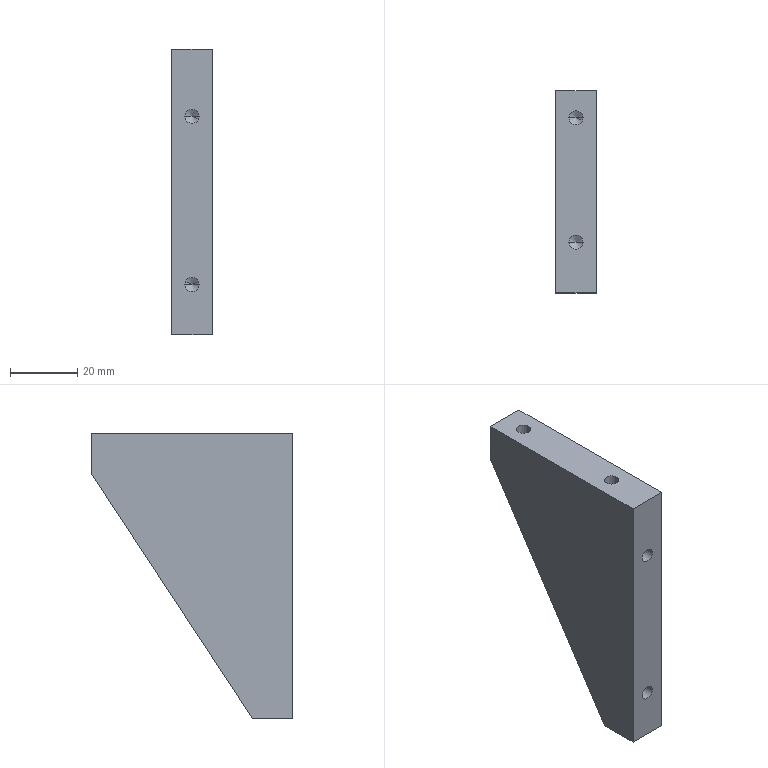Component | SolidWorks | HandlingMechanism-2_A0111-2 | 1 solid | 23 faces | box 12 x 60 x 85 mm | volume 39377 mm3 | cylinder 8 | cone 8 | plane 7 | commonest cylinder face diameters 4.2 x8
build123d program:
from build123d import *

# Parameters (mm, degrees)
SKETCH1_W             = 85
SKETCH1_H             = 60
BOSS_EXTRUDE1_DEPTH   = 6
CUT_EXTRUDE1_DEPTH    = 12
M5_TAPPED_HOLE1_D     = 4.2
M5_TAPPED_HOLE1_DEPTH = 14
M5_TAPPED_HOLE1_TIP   = 1.262
M5_TAPPED_HOLE2_D     = 4.2
M5_TAPPED_HOLE2_DEPTH = 14
M5_TAPPED_HOLE2_TIP   = 1.262


with BuildPart() as part:
    # Sketch1 → Boss-Extrude1 (new, symmetric)
    with BuildSketch(Plane.XY):
        Rectangle(SKETCH1_W, SKETCH1_H)
    extrude(amount=BOSS_EXTRUDE1_DEPTH, both=True)

    # Sketch2 → Cut-Extrude1 (cut)
    with BuildSketch(Plane.XY.offset(6)):
        Polygon((-42.5, -18), (30.5, 30), (-42.5, 30), align=None)
    extrude(amount=-CUT_EXTRUDE1_DEPTH, mode=Mode.SUBTRACT)

    # M5 Tapped Hole1
    with Locations(Plane(origin=(0, -30, 0), x_dir=(-1, 0, 0), z_dir=(0, -1, 0))):
        with Locations((27.5, 0), (-22.5, 0)):
            Hole(M5_TAPPED_HOLE1_D / 2, depth=M5_TAPPED_HOLE1_DEPTH)
            with Locations((0, 0, -(M5_TAPPED_HOLE1_DEPTH + M5_TAPPED_HOLE1_TIP / 2))):  # 118° drill point
                Cone(0, M5_TAPPED_HOLE1_D / 2, M5_TAPPED_HOLE1_TIP, mode=Mode.SUBTRACT)

    # M5 Tapped Hole2
    with Locations(Plane(origin=(42.5, 0, 0), x_dir=(0, 0, -1), z_dir=(1, 0, 0))):
        with Locations((0, 22), (0, -15)):
            Hole(M5_TAPPED_HOLE2_D / 2, depth=M5_TAPPED_HOLE2_DEPTH)
            with Locations((0, 0, -(M5_TAPPED_HOLE2_DEPTH + M5_TAPPED_HOLE2_TIP / 2))):  # 118° drill point
                Cone(0, M5_TAPPED_HOLE2_D / 2, M5_TAPPED_HOLE2_TIP, mode=Mode.SUBTRACT)


solid = part.part

# Placed as in the assembly
solid = solid.moved(Location((25.881, 81.5, 80.5), (0, -90, 0)))
STEP:
#1=COLOUR_RGB('',0.7922,0.8196,0.9333);
#2=FILL_AREA_STYLE_COLOUR('',#1);
#3=FILL_AREA_STYLE('',(#2));
#4=SURFACE_STYLE_FILL_AREA(#3);
#5=SURFACE_SIDE_STYLE('',(#4));
#6=SURFACE_STYLE_USAGE(.BOTH.,#5);
#7=PRESENTATION_STYLE_ASSIGNMENT((#6));
#8=CARTESIAN_POINT('',(0.9362,4.075,4.291));
#9=VERTEX_POINT('',#8);
#10=CARTESIAN_POINT('',(1.102,4.075,4.291));
#11=VERTEX_POINT('',#10);
#12=CARTESIAN_POINT('',(1.019,4.075,4.291));
#13=DIRECTION('',(0.,-0.,1.));
#14=DIRECTION('',(1.,0.,-0.));
#15=AXIS2_PLACEMENT_3D('',#12,#13,#14);
#16=CIRCLE('',#15,0.08268);
#17=EDGE_CURVE('',#9,#11,#16,.T.);
#18=ORIENTED_EDGE('',*,*,#17,.F.);
#19=CARTESIAN_POINT('',(0.9362,4.075,4.843));
#20=VERTEX_POINT('',#19);
#21=CARTESIAN_POINT('',(0.9362,4.075,4.843));
#22=DIRECTION('',(0.,-0.,1.));
#23=VECTOR('',#22,39.37);
#24=LINE('',#21,#23);
#25=EDGE_CURVE('',#9,#20,#24,.T.);
#26=ORIENTED_EDGE('',*,*,#25,.T.);
#27=CARTESIAN_POINT('',(1.102,4.075,4.843));
#28=VERTEX_POINT('',#27);
#29=CARTESIAN_POINT('',(1.019,4.075,4.843));
#30=DIRECTION('',(0.,-0.,1.));
#31=DIRECTION('',(1.,0.,-0.));
#32=AXIS2_PLACEMENT_3D('',#29,#30,#31);
#33=CIRCLE('',#32,0.08268);
#34=EDGE_CURVE('',#20,#28,#33,.T.);
#35=ORIENTED_EDGE('',*,*,#34,.T.);
#36=CARTESIAN_POINT('',(1.102,4.075,4.843));
#37=DIRECTION('',(0.,-0.,1.));
#38=VECTOR('',#37,39.37);
#39=LINE('',#36,#38);
#40=EDGE_CURVE('',#11,#28,#39,.T.);
#41=ORIENTED_EDGE('',*,*,#40,.F.);
#42=EDGE_LOOP('',(#18,#26,#35,#41));
#43=FACE_OUTER_BOUND('',#42,.T.);
#44=CARTESIAN_POINT('',(1.019,4.075,4.843));
#45=DIRECTION('',(0.,-0.,1.));
#46=DIRECTION('',(1.,0.,-0.));
#47=AXIS2_PLACEMENT_3D('',#44,#45,#46);
#48=CYLINDRICAL_SURFACE('',#47,0.08268);
#49=ADVANCED_FACE('',(#43),#48,.F.);
#50=CARTESIAN_POINT('',(1.019,4.075,4.242));
#51=VERTEX_POINT('',#50);
#52=CARTESIAN_POINT('',(1.102,4.075,4.291));
#53=DIRECTION('',(0.8572,0.,0.515));
#54=VECTOR('',#53,39.37);
#55=LINE('',#52,#54);
#56=EDGE_CURVE('',#51,#11,#55,.T.);
#57=ORIENTED_EDGE('',*,*,#56,.F.);
#58=CARTESIAN_POINT('',(0.9362,4.075,4.291));
#59=DIRECTION('',(-0.8572,-0.,0.515));
#60=VECTOR('',#59,39.37);
#61=LINE('',#58,#60);
#62=EDGE_CURVE('',#51,#9,#61,.T.);
#63=ORIENTED_EDGE('',*,*,#62,.T.);
#64=ORIENTED_EDGE('',*,*,#17,.T.);
#65=EDGE_LOOP('',(#57,#63,#64));
#66=FACE_OUTER_BOUND('',#65,.T.);
#67=CARTESIAN_POINT('',(1.019,4.075,4.291));
#68=DIRECTION('',(0.,-0.,1.));
#69=DIRECTION('',(1.,0.,-0.));
#70=AXIS2_PLACEMENT_3D('',#67,#68,#69);
#71=CONICAL_SURFACE('',#70,0.08268,1.03);
#72=ADVANCED_FACE('',(#66),#71,.F.);
#73=CARTESIAN_POINT('',(0.9362,2.618,4.291));
#74=VERTEX_POINT('',#73);
#75=CARTESIAN_POINT('',(1.102,2.618,4.291));
#76=VERTEX_POINT('',#75);
#77=CARTESIAN_POINT('',(1.019,2.618,4.291));
#78=DIRECTION('',(0.,-0.,1.));
#79=DIRECTION('',(1.,0.,-0.));
#80=AXIS2_PLACEMENT_3D('',#77,#78,#79);
#81=CIRCLE('',#80,0.08268);
#82=EDGE_CURVE('',#74,#76,#81,.T.);
#83=ORIENTED_EDGE('',*,*,#82,.F.);
#84=CARTESIAN_POINT('',(0.9362,2.618,4.843));
#85=VERTEX_POINT('',#84);
#86=CARTESIAN_POINT('',(0.9362,2.618,4.843));
#87=DIRECTION('',(0.,-0.,1.));
#88=VECTOR('',#87,39.37);
#89=LINE('',#86,#88);
#90=EDGE_CURVE('',#74,#85,#89,.T.);
#91=ORIENTED_EDGE('',*,*,#90,.T.);
#92=CARTESIAN_POINT('',(1.102,2.618,4.843));
#93=VERTEX_POINT('',#92);
#94=CARTESIAN_POINT('',(1.019,2.618,4.843));
#95=DIRECTION('',(0.,-0.,1.));
#96=DIRECTION('',(1.,0.,-0.));
#97=AXIS2_PLACEMENT_3D('',#94,#95,#96);
#98=CIRCLE('',#97,0.08268);
#99=EDGE_CURVE('',#85,#93,#98,.T.);
#100=ORIENTED_EDGE('',*,*,#99,.T.);
#101=CARTESIAN_POINT('',(1.102,2.618,4.843));
#102=DIRECTION('',(0.,-0.,1.));
#103=VECTOR('',#102,39.37);
#104=LINE('',#101,#103);
#105=EDGE_CURVE('',#76,#93,#104,.T.);
#106=ORIENTED_EDGE('',*,*,#105,.F.);
#107=EDGE_LOOP('',(#83,#91,#100,#106));
#108=FACE_OUTER_BOUND('',#107,.T.);
#109=CARTESIAN_POINT('',(1.019,2.618,4.843));
#110=DIRECTION('',(0.,-0.,1.));
#111=DIRECTION('',(1.,0.,-0.));
#112=AXIS2_PLACEMENT_3D('',#109,#110,#111);
#113=CYLINDRICAL_SURFACE('',#112,0.08268);
#114=ADVANCED_FACE('',(#108),#113,.F.);
#115=CARTESIAN_POINT('',(1.019,2.618,4.242));
#116=VERTEX_POINT('',#115);
#117=CARTESIAN_POINT('',(1.102,2.618,4.291));
#118=DIRECTION('',(0.8572,0.,0.515));
#119=VECTOR('',#118,39.37);
#120=LINE('',#117,#119);
#121=EDGE_CURVE('',#116,#76,#120,.T.);
#122=ORIENTED_EDGE('',*,*,#121,.F.);
#123=CARTESIAN_POINT('',(0.9362,2.618,4.291));
#124=DIRECTION('',(-0.8572,-0.,0.515));
#125=VECTOR('',#124,39.37);
#126=LINE('',#123,#125);
#127=EDGE_CURVE('',#116,#74,#126,.T.);
#128=ORIENTED_EDGE('',*,*,#127,.T.);
#129=ORIENTED_EDGE('',*,*,#82,.T.);
#130=EDGE_LOOP('',(#122,#128,#129));
#131=FACE_OUTER_BOUND('',#130,.T.);
#132=CARTESIAN_POINT('',(1.019,2.618,4.291));
#133=DIRECTION('',(0.,-0.,1.));
#134=DIRECTION('',(1.,0.,-0.));
#135=AXIS2_PLACEMENT_3D('',#132,#133,#134);
#136=CONICAL_SURFACE('',#135,0.08268,1.03);
#137=ADVANCED_FACE('',(#131),#136,.F.);
#138=CARTESIAN_POINT('',(0.9362,2.579,2.087));
#139=VERTEX_POINT('',#138);
#140=CARTESIAN_POINT('',(1.102,2.579,2.087));
#141=VERTEX_POINT('',#140);
#142=CARTESIAN_POINT('',(1.019,2.579,2.087));
#143=DIRECTION('',(0.,-1.,-0.));
#144=DIRECTION('',(1.,0.,-0.));
#145=AXIS2_PLACEMENT_3D('',#142,#143,#144);
#146=CIRCLE('',#145,0.08268);
#147=EDGE_CURVE('',#139,#141,#146,.T.);
#148=ORIENTED_EDGE('',*,*,#147,.F.);
#149=CARTESIAN_POINT('',(0.9362,2.028,2.087));
#150=VERTEX_POINT('',#149);
#151=CARTESIAN_POINT('',(0.9362,2.028,2.087));
#152=DIRECTION('',(0.,-1.,-0.));
#153=VECTOR('',#152,39.37);
#154=LINE('',#151,#153);
#155=EDGE_CURVE('',#139,#150,#154,.T.);
#156=ORIENTED_EDGE('',*,*,#155,.T.);
#157=CARTESIAN_POINT('',(1.102,2.028,2.087));
#158=VERTEX_POINT('',#157);
#159=CARTESIAN_POINT('',(1.019,2.028,2.087));
#160=DIRECTION('',(0.,-1.,-0.));
#161=DIRECTION('',(1.,0.,-0.));
#162=AXIS2_PLACEMENT_3D('',#159,#160,#161);
#163=CIRCLE('',#162,0.08268);
#164=EDGE_CURVE('',#150,#158,#163,.T.);
#165=ORIENTED_EDGE('',*,*,#164,.T.);
#166=CARTESIAN_POINT('',(1.102,2.028,2.087));
#167=DIRECTION('',(0.,-1.,-0.));
#168=VECTOR('',#167,39.37);
#169=LINE('',#166,#168);
#170=EDGE_CURVE('',#141,#158,#169,.T.);
#171=ORIENTED_EDGE('',*,*,#170,.F.);
#172=EDGE_LOOP('',(#148,#156,#165,#171));
#173=FACE_OUTER_BOUND('',#172,.T.);
#174=CARTESIAN_POINT('',(1.019,2.028,2.087));
#175=DIRECTION('',(0.,-1.,-0.));
#176=DIRECTION('',(1.,0.,-0.));
#177=AXIS2_PLACEMENT_3D('',#174,#175,#176);
#178=CYLINDRICAL_SURFACE('',#177,0.08268);
#179=ADVANCED_FACE('',(#173),#178,.F.);
#180=CARTESIAN_POINT('',(1.019,2.628,2.087));
#181=VERTEX_POINT('',#180);
#182=CARTESIAN_POINT('',(1.102,2.579,2.087));
#183=DIRECTION('',(0.8572,-0.515,-0.));
#184=VECTOR('',#183,39.37);
#185=LINE('',#182,#184);
#186=EDGE_CURVE('',#181,#141,#185,.T.);
#187=ORIENTED_EDGE('',*,*,#186,.F.);
#188=CARTESIAN_POINT('',(0.9362,2.579,2.087));
#189=DIRECTION('',(-0.8572,-0.515,0.));
#190=VECTOR('',#189,39.37);
#191=LINE('',#188,#190);
#192=EDGE_CURVE('',#181,#139,#191,.T.);
#193=ORIENTED_EDGE('',*,*,#192,.T.);
#194=ORIENTED_EDGE('',*,*,#147,.T.);
#195=EDGE_LOOP('',(#187,#193,#194));
#196=FACE_OUTER_BOUND('',#195,.T.);
#197=CARTESIAN_POINT('',(1.019,2.579,2.087));
#198=DIRECTION('',(0.,-1.,-0.));
#199=DIRECTION('',(1.,0.,-0.));
#200=AXIS2_PLACEMENT_3D('',#197,#198,#199);
#201=CONICAL_SURFACE('',#200,0.08268,1.03);
#202=ADVANCED_FACE('',(#196),#201,.F.);
#203=CARTESIAN_POINT('',(0.9362,2.579,4.055));
#204=VERTEX_POINT('',#203);
#205=CARTESIAN_POINT('',(1.102,2.579,4.055));
#206=VERTEX_POINT('',#205);
#207=CARTESIAN_POINT('',(1.019,2.579,4.055));
#208=DIRECTION('',(0.,-1.,-0.));
#209=DIRECTION('',(1.,0.,-0.));
#210=AXIS2_PLACEMENT_3D('',#207,#208,#209);
#211=CIRCLE('',#210,0.08268);
#212=EDGE_CURVE('',#204,#206,#211,.T.);
#213=ORIENTED_EDGE('',*,*,#212,.F.);
#214=CARTESIAN_POINT('',(0.9362,2.028,4.055));
#215=VERTEX_POINT('',#214);
#216=CARTESIAN_POINT('',(0.9362,2.028,4.055));
#217=DIRECTION('',(0.,-1.,-0.));
#218=VECTOR('',#217,39.37);
#219=LINE('',#216,#218);
#220=EDGE_CURVE('',#204,#215,#219,.T.);
#221=ORIENTED_EDGE('',*,*,#220,.T.);
#222=CARTESIAN_POINT('',(1.102,2.028,4.055));
#223=VERTEX_POINT('',#222);
#224=CARTESIAN_POINT('',(1.019,2.028,4.055));
#225=DIRECTION('',(0.,-1.,-0.));
#226=DIRECTION('',(1.,0.,-0.));
#227=AXIS2_PLACEMENT_3D('',#224,#225,#226);
#228=CIRCLE('',#227,0.08268);
#229=EDGE_CURVE('',#215,#223,#228,.T.);
#230=ORIENTED_EDGE('',*,*,#229,.T.);
#231=CARTESIAN_POINT('',(1.102,2.028,4.055));
#232=DIRECTION('',(0.,-1.,-0.));
#233=VECTOR('',#232,39.37);
#234=LINE('',#231,#233);
#235=EDGE_CURVE('',#206,#223,#234,.T.);
#236=ORIENTED_EDGE('',*,*,#235,.F.);
#237=EDGE_LOOP('',(#213,#221,#230,#236));
#238=FACE_OUTER_BOUND('',#237,.T.);
#239=CARTESIAN_POINT('',(1.019,2.028,4.055));
#240=DIRECTION('',(0.,-1.,-0.));
#241=DIRECTION('',(1.,0.,-0.));
#242=AXIS2_PLACEMENT_3D('',#239,#240,#241);
#243=CYLINDRICAL_SURFACE('',#242,0.08268);
#244=ADVANCED_FACE('',(#238),#243,.F.);
#245=CARTESIAN_POINT('',(1.019,2.628,4.055));
#246=VERTEX_POINT('',#245);
#247=CARTESIAN_POINT('',(1.102,2.579,4.055));
#248=DIRECTION('',(0.8572,-0.515,-0.));
#249=VECTOR('',#248,39.37);
#250=LINE('',#247,#249);
#251=EDGE_CURVE('',#246,#206,#250,.T.);
#252=ORIENTED_EDGE('',*,*,#251,.F.);
#253=CARTESIAN_POINT('',(0.9362,2.579,4.055));
#254=DIRECTION('',(-0.8572,-0.515,0.));
#255=VECTOR('',#254,39.37);
#256=LINE('',#253,#255);
#257=EDGE_CURVE('',#246,#204,#256,.T.);
#258=ORIENTED_EDGE('',*,*,#257,.T.);
#259=ORIENTED_EDGE('',*,*,#212,.T.);
#260=EDGE_LOOP('',(#252,#258,#259));
#261=FACE_OUTER_BOUND('',#260,.T.);
#262=CARTESIAN_POINT('',(1.019,2.579,4.055));
#263=DIRECTION('',(0.,-1.,-0.));
#264=DIRECTION('',(1.,0.,-0.));
#265=AXIS2_PLACEMENT_3D('',#262,#263,#264);
#266=CONICAL_SURFACE('',#265,0.08268,1.03);
#267=ADVANCED_FACE('',(#261),#266,.F.);
#268=CARTESIAN_POINT('',(1.019,4.075,4.843));
#269=DIRECTION('',(0.,-0.,1.));
#270=DIRECTION('',(1.,0.,-0.));
#271=AXIS2_PLACEMENT_3D('',#268,#269,#270);
#272=CIRCLE('',#271,0.08268);
#273=EDGE_CURVE('',#28,#20,#272,.T.);
#274=ORIENTED_EDGE('',*,*,#273,.F.);
#275=ORIENTED_EDGE('',*,*,#34,.F.);
#276=EDGE_LOOP('',(#274,#275));
#277=FACE_BOUND('',#276,.T.);
#278=CARTESIAN_POINT('',(1.019,2.618,4.843));
#279=DIRECTION('',(0.,-0.,1.));
#280=DIRECTION('',(1.,0.,-0.));
#281=AXIS2_PLACEMENT_3D('',#278,#279,#280);
#282=CIRCLE('',#281,0.08268);
#283=EDGE_CURVE('',#93,#85,#282,.T.);
#284=ORIENTED_EDGE('',*,*,#283,.F.);
#285=ORIENTED_EDGE('',*,*,#99,.F.);
#286=EDGE_LOOP('',(#284,#285));
#287=FACE_BOUND('',#286,.T.);
#288=CARTESIAN_POINT('',(1.255,2.028,4.843));
#289=VERTEX_POINT('',#288);
#290=CARTESIAN_POINT('',(1.255,4.39,4.843));
#291=VERTEX_POINT('',#290);
#292=CARTESIAN_POINT('',(1.255,4.39,4.843));
#293=DIRECTION('',(-0.,1.,0.));
#294=VECTOR('',#293,39.37);
#295=LINE('',#292,#294);
#296=EDGE_CURVE('',#289,#291,#295,.T.);
#297=ORIENTED_EDGE('',*,*,#296,.T.);
#298=CARTESIAN_POINT('',(0.7827,4.39,4.843));
#299=VERTEX_POINT('',#298);
#300=CARTESIAN_POINT('',(0.7827,4.39,4.843));
#301=DIRECTION('',(1.,0.,-0.));
#302=VECTOR('',#301,39.37);
#303=LINE('',#300,#302);
#304=EDGE_CURVE('',#299,#291,#303,.T.);
#305=ORIENTED_EDGE('',*,*,#304,.F.);
#306=CARTESIAN_POINT('',(0.7827,2.028,4.843));
#307=VERTEX_POINT('',#306);
#308=CARTESIAN_POINT('',(0.7827,4.39,4.843));
#309=DIRECTION('',(-0.,1.,0.));
#310=VECTOR('',#309,39.37);
#311=LINE('',#308,#310);
#312=EDGE_CURVE('',#307,#299,#311,.T.);
#313=ORIENTED_EDGE('',*,*,#312,.F.);
#314=CARTESIAN_POINT('',(0.7827,2.028,4.843));
#315=DIRECTION('',(1.,0.,-0.));
#316=VECTOR('',#315,39.37);
#317=LINE('',#314,#316);
#318=EDGE_CURVE('',#307,#289,#317,.T.);
#319=ORIENTED_EDGE('',*,*,#318,.T.);
#320=EDGE_LOOP('',(#297,#305,#313,#319));
#321=FACE_OUTER_BOUND('',#320,.T.);
#322=CARTESIAN_POINT('',(0.7827,4.39,4.843));
#323=DIRECTION('',(-0.,0.,-1.));
#324=DIRECTION('',(0.,-1.,-0.));
#325=AXIS2_PLACEMENT_3D('',#322,#323,#324);
#326=PLANE('',#325);
#327=ADVANCED_FACE('',(#277,#287,#321),#326,.F.);
#328=CARTESIAN_POINT('',(1.255,4.39,4.37));
#329=VERTEX_POINT('',#328);
#330=CARTESIAN_POINT('',(1.255,4.39,1.496));
#331=DIRECTION('',(-0.,0.,-1.));
#332=VECTOR('',#331,39.37);
#333=LINE('',#330,#332);
#334=EDGE_CURVE('',#291,#329,#333,.T.);
#335=ORIENTED_EDGE('',*,*,#334,.T.);
#336=CARTESIAN_POINT('',(0.7827,4.39,4.37));
#337=VERTEX_POINT('',#336);
#338=CARTESIAN_POINT('',(1.255,4.39,4.37));
#339=DIRECTION('',(-1.,-0.,0.));
#340=VECTOR('',#339,39.37);
#341=LINE('',#338,#340);
#342=EDGE_CURVE('',#329,#337,#341,.T.);
#343=ORIENTED_EDGE('',*,*,#342,.T.);
#344=CARTESIAN_POINT('',(0.7827,4.39,1.496));
#345=DIRECTION('',(-0.,0.,-1.));
#346=VECTOR('',#345,39.37);
#347=LINE('',#344,#346);
#348=EDGE_CURVE('',#299,#337,#347,.T.);
#349=ORIENTED_EDGE('',*,*,#348,.F.);
#350=ORIENTED_EDGE('',*,*,#304,.T.);
#351=EDGE_LOOP('',(#335,#343,#349,#350));
#352=FACE_OUTER_BOUND('',#351,.T.);
#353=CARTESIAN_POINT('',(0.7827,4.39,1.496));
#354=DIRECTION('',(0.,-1.,-0.));
#355=DIRECTION('',(1.,0.,-0.));
#356=AXIS2_PLACEMENT_3D('',#353,#354,#355);
#357=PLANE('',#356);
#358=ADVANCED_FACE('',(#352),#357,.F.);
#359=CARTESIAN_POINT('',(0.7827,2.5,1.496));
#360=VERTEX_POINT('',#359);
#361=CARTESIAN_POINT('',(0.7827,2.028,1.496));
#362=VERTEX_POINT('',#361);
#363=CARTESIAN_POINT('',(0.7827,4.39,1.496));
#364=DIRECTION('',(0.,-1.,-0.));
#365=VECTOR('',#364,39.37);
#366=LINE('',#363,#365);
#367=EDGE_CURVE('',#360,#362,#366,.T.);
#368=ORIENTED_EDGE('',*,*,#367,.F.);
#369=CARTESIAN_POINT('',(1.255,2.5,1.496));
#370=VERTEX_POINT('',#369);
#371=CARTESIAN_POINT('',(1.255,2.5,1.496));
#372=DIRECTION('',(-1.,-0.,0.));
#373=VECTOR('',#372,39.37);
#374=LINE('',#371,#373);
#375=EDGE_CURVE('',#370,#360,#374,.T.);
#376=ORIENTED_EDGE('',*,*,#375,.F.);
#377=CARTESIAN_POINT('',(1.255,2.028,1.496));
#378=VERTEX_POINT('',#377);
#379=CARTESIAN_POINT('',(1.255,4.39,1.496));
#380=DIRECTION('',(0.,-1.,-0.));
#381=VECTOR('',#380,39.37);
#382=LINE('',#379,#381);
#383=EDGE_CURVE('',#370,#378,#382,.T.);
#384=ORIENTED_EDGE('',*,*,#383,.T.);
#385=CARTESIAN_POINT('',(0.7827,2.028,1.496));
#386=DIRECTION('',(1.,0.,-0.));
#387=VECTOR('',#386,39.37);
#388=LINE('',#385,#387);
#389=EDGE_CURVE('',#362,#378,#388,.T.);
#390=ORIENTED_EDGE('',*,*,#389,.F.);
#391=EDGE_LOOP('',(#368,#376,#384,#390));
#392=FACE_OUTER_BOUND('',#391,.T.);
#393=CARTESIAN_POINT('',(0.7827,4.39,1.496));
#394=DIRECTION('',(0.,-0.,1.));
#395=DIRECTION('',(-0.,1.,0.));
#396=AXIS2_PLACEMENT_3D('',#393,#394,#395);
#397=PLANE('',#396);
#398=ADVANCED_FACE('',(#392),#397,.F.);
#399=CARTESIAN_POINT('',(1.019,2.028,2.087));
#400=DIRECTION('',(0.,-1.,-0.));
#401=DIRECTION('',(1.,0.,-0.));
#402=AXIS2_PLACEMENT_3D('',#399,#400,#401);
#403=CIRCLE('',#402,0.08268);
#404=EDGE_CURVE('',#158,#150,#403,.T.);
#405=ORIENTED_EDGE('',*,*,#404,.F.);
#406=ORIENTED_EDGE('',*,*,#164,.F.);
#407=EDGE_LOOP('',(#405,#406));
#408=FACE_BOUND('',#407,.T.);
#409=CARTESIAN_POINT('',(1.019,2.028,4.055));
#410=DIRECTION('',(0.,-1.,-0.));
#411=DIRECTION('',(1.,0.,-0.));
#412=AXIS2_PLACEMENT_3D('',#409,#410,#411);
#413=CIRCLE('',#412,0.08268);
#414=EDGE_CURVE('',#223,#215,#413,.T.);
#415=ORIENTED_EDGE('',*,*,#414,.F.);
#416=ORIENTED_EDGE('',*,*,#229,.F.);
#417=EDGE_LOOP('',(#415,#416));
#418=FACE_BOUND('',#417,.T.);
#419=CARTESIAN_POINT('',(1.255,2.028,1.496));
#420=DIRECTION('',(0.,-0.,1.));
#421=VECTOR('',#420,39.37);
#422=LINE('',#419,#421);
#423=EDGE_CURVE('',#378,#289,#422,.T.);
#424=ORIENTED_EDGE('',*,*,#423,.T.);
#425=ORIENTED_EDGE('',*,*,#318,.F.);
#426=CARTESIAN_POINT('',(0.7827,2.028,1.496));
#427=DIRECTION('',(0.,-0.,1.));
#428=VECTOR('',#427,39.37);
#429=LINE('',#426,#428);
#430=EDGE_CURVE('',#362,#307,#429,.T.);
#431=ORIENTED_EDGE('',*,*,#430,.F.);
#432=ORIENTED_EDGE('',*,*,#389,.T.);
#433=EDGE_LOOP('',(#424,#425,#431,#432));
#434=FACE_OUTER_BOUND('',#433,.T.);
#435=CARTESIAN_POINT('',(0.7827,2.028,1.496));
#436=DIRECTION('',(-0.,1.,0.));
#437=DIRECTION('',(-1.,-0.,0.));
#438=AXIS2_PLACEMENT_3D('',#435,#436,#437);
#439=PLANE('',#438);
#440=ADVANCED_FACE('',(#408,#418,#434),#439,.F.);
#441=CARTESIAN_POINT('',(0.7827,2.5,1.496));
#442=DIRECTION('',(0.,0.5494,0.8356));
#443=VECTOR('',#442,39.37);
#444=LINE('',#441,#443);
#445=EDGE_CURVE('',#360,#337,#444,.T.);
#446=ORIENTED_EDGE('',*,*,#445,.F.);
#447=ORIENTED_EDGE('',*,*,#367,.T.);
#448=ORIENTED_EDGE('',*,*,#430,.T.);
#449=ORIENTED_EDGE('',*,*,#312,.T.);
#450=ORIENTED_EDGE('',*,*,#348,.T.);
#451=EDGE_LOOP('',(#446,#447,#448,#449,#450));
#452=FACE_OUTER_BOUND('',#451,.T.);
#453=CARTESIAN_POINT('',(0.7827,3.209,3.169));
#454=DIRECTION('',(-1.,-0.,0.));
#455=DIRECTION('',(0.,-0.,1.));
#456=AXIS2_PLACEMENT_3D('',#453,#454,#455);
#457=PLANE('',#456);
#458=ADVANCED_FACE('',(#452),#457,.T.);
#459=ORIENTED_EDGE('',*,*,#383,.F.);
#460=CARTESIAN_POINT('',(1.255,2.5,1.496));
#461=DIRECTION('',(0.,0.5494,0.8356));
#462=VECTOR('',#461,39.37);
#463=LINE('',#460,#462);
#464=EDGE_CURVE('',#370,#329,#463,.T.);
#465=ORIENTED_EDGE('',*,*,#464,.T.);
#466=ORIENTED_EDGE('',*,*,#334,.F.);
#467=ORIENTED_EDGE('',*,*,#296,.F.);
#468=ORIENTED_EDGE('',*,*,#423,.F.);
#469=EDGE_LOOP('',(#459,#465,#466,#467,#468));
#470=FACE_OUTER_BOUND('',#469,.T.);
#471=CARTESIAN_POINT('',(1.255,3.209,3.169));
#472=DIRECTION('',(-1.,-0.,0.));
#473=DIRECTION('',(0.,-0.,1.));
#474=AXIS2_PLACEMENT_3D('',#471,#472,#473);
#475=PLANE('',#474);
#476=ADVANCED_FACE('',(#470),#475,.F.);
#477=ORIENTED_EDGE('',*,*,#445,.T.);
#478=ORIENTED_EDGE('',*,*,#342,.F.);
#479=ORIENTED_EDGE('',*,*,#464,.F.);
#480=ORIENTED_EDGE('',*,*,#375,.T.);
#481=EDGE_LOOP('',(#477,#478,#479,#480));
#482=FACE_OUTER_BOUND('',#481,.T.);
#483=CARTESIAN_POINT('',(1.255,2.5,1.496));
#484=DIRECTION('',(0.,-0.8356,0.5494));
#485=DIRECTION('',(0.,0.5494,0.8356));
#486=AXIS2_PLACEMENT_3D('',#483,#484,#485);
#487=PLANE('',#486);
#488=ADVANCED_FACE('',(#482),#487,.F.);
#489=ORIENTED_EDGE('',*,*,#257,.F.);
#490=ORIENTED_EDGE('',*,*,#251,.T.);
#491=CARTESIAN_POINT('',(1.019,2.579,4.055));
#492=DIRECTION('',(0.,-1.,-0.));
#493=DIRECTION('',(1.,0.,-0.));
#494=AXIS2_PLACEMENT_3D('',#491,#492,#493);
#495=CIRCLE('',#494,0.08268);
#496=EDGE_CURVE('',#206,#204,#495,.T.);
#497=ORIENTED_EDGE('',*,*,#496,.T.);
#498=EDGE_LOOP('',(#489,#490,#497));
#499=FACE_OUTER_BOUND('',#498,.T.);
#500=CARTESIAN_POINT('',(1.019,2.579,4.055));
#501=DIRECTION('',(0.,-1.,-0.));
#502=DIRECTION('',(1.,0.,-0.));
#503=AXIS2_PLACEMENT_3D('',#500,#501,#502);
#504=CONICAL_SURFACE('',#503,0.08268,1.03);
#505=ADVANCED_FACE('',(#499),#504,.F.);
#506=ORIENTED_EDGE('',*,*,#220,.F.);
#507=ORIENTED_EDGE('',*,*,#496,.F.);
#508=ORIENTED_EDGE('',*,*,#235,.T.);
#509=ORIENTED_EDGE('',*,*,#414,.T.);
#510=EDGE_LOOP('',(#506,#507,#508,#509));
#511=FACE_OUTER_BOUND('',#510,.T.);
#512=CARTESIAN_POINT('',(1.019,2.028,4.055));
#513=DIRECTION('',(0.,-1.,-0.));
#514=DIRECTION('',(1.,0.,-0.));
#515=AXIS2_PLACEMENT_3D('',#512,#513,#514);
#516=CYLINDRICAL_SURFACE('',#515,0.08268);
#517=ADVANCED_FACE('',(#511),#516,.F.);
#518=ORIENTED_EDGE('',*,*,#192,.F.);
#519=ORIENTED_EDGE('',*,*,#186,.T.);
#520=CARTESIAN_POINT('',(1.019,2.579,2.087));
#521=DIRECTION('',(0.,-1.,-0.));
#522=DIRECTION('',(1.,0.,-0.));
#523=AXIS2_PLACEMENT_3D('',#520,#521,#522);
#524=CIRCLE('',#523,0.08268);
#525=EDGE_CURVE('',#141,#139,#524,.T.);
#526=ORIENTED_EDGE('',*,*,#525,.T.);
#527=EDGE_LOOP('',(#518,#519,#526));
#528=FACE_OUTER_BOUND('',#527,.T.);
#529=CARTESIAN_POINT('',(1.019,2.579,2.087));
#530=DIRECTION('',(0.,-1.,-0.));
#531=DIRECTION('',(1.,0.,-0.));
#532=AXIS2_PLACEMENT_3D('',#529,#530,#531);
#533=CONICAL_SURFACE('',#532,0.08268,1.03);
#534=ADVANCED_FACE('',(#528),#533,.F.);
#535=ORIENTED_EDGE('',*,*,#155,.F.);
#536=ORIENTED_EDGE('',*,*,#525,.F.);
#537=ORIENTED_EDGE('',*,*,#170,.T.);
#538=ORIENTED_EDGE('',*,*,#404,.T.);
#539=EDGE_LOOP('',(#535,#536,#537,#538));
#540=FACE_OUTER_BOUND('',#539,.T.);
#541=CARTESIAN_POINT('',(1.019,2.028,2.087));
#542=DIRECTION('',(0.,-1.,-0.));
#543=DIRECTION('',(1.,0.,-0.));
#544=AXIS2_PLACEMENT_3D('',#541,#542,#543);
#545=CYLINDRICAL_SURFACE('',#544,0.08268);
#546=ADVANCED_FACE('',(#540),#545,.F.);
#547=ORIENTED_EDGE('',*,*,#127,.F.);
#548=ORIENTED_EDGE('',*,*,#121,.T.);
#549=CARTESIAN_POINT('',(1.019,2.618,4.291));
#550=DIRECTION('',(0.,-0.,1.));
#551=DIRECTION('',(1.,0.,-0.));
#552=AXIS2_PLACEMENT_3D('',#549,#550,#551);
#553=CIRCLE('',#552,0.08268);
#554=EDGE_CURVE('',#76,#74,#553,.T.);
#555=ORIENTED_EDGE('',*,*,#554,.T.);
#556=EDGE_LOOP('',(#547,#548,#555));
#557=FACE_OUTER_BOUND('',#556,.T.);
#558=CARTESIAN_POINT('',(1.019,2.618,4.291));
#559=DIRECTION('',(0.,-0.,1.));
#560=DIRECTION('',(1.,0.,-0.));
#561=AXIS2_PLACEMENT_3D('',#558,#559,#560);
#562=CONICAL_SURFACE('',#561,0.08268,1.03);
#563=ADVANCED_FACE('',(#557),#562,.F.);
#564=ORIENTED_EDGE('',*,*,#90,.F.);
#565=ORIENTED_EDGE('',*,*,#554,.F.);
#566=ORIENTED_EDGE('',*,*,#105,.T.);
#567=ORIENTED_EDGE('',*,*,#283,.T.);
#568=EDGE_LOOP('',(#564,#565,#566,#567));
#569=FACE_OUTER_BOUND('',#568,.T.);
#570=CARTESIAN_POINT('',(1.019,2.618,4.843));
#571=DIRECTION('',(0.,-0.,1.));
#572=DIRECTION('',(1.,0.,-0.));
#573=AXIS2_PLACEMENT_3D('',#570,#571,#572);
#574=CYLINDRICAL_SURFACE('',#573,0.08268);
#575=ADVANCED_FACE('',(#569),#574,.F.);
#576=ORIENTED_EDGE('',*,*,#62,.F.);
#577=ORIENTED_EDGE('',*,*,#56,.T.);
#578=CARTESIAN_POINT('',(1.019,4.075,4.291));
#579=DIRECTION('',(0.,-0.,1.));
#580=DIRECTION('',(1.,0.,-0.));
#581=AXIS2_PLACEMENT_3D('',#578,#579,#580);
#582=CIRCLE('',#581,0.08268);
#583=EDGE_CURVE('',#11,#9,#582,.T.);
#584=ORIENTED_EDGE('',*,*,#583,.T.);
#585=EDGE_LOOP('',(#576,#577,#584));
#586=FACE_OUTER_BOUND('',#585,.T.);
#587=CARTESIAN_POINT('',(1.019,4.075,4.291));
#588=DIRECTION('',(0.,-0.,1.));
#589=DIRECTION('',(1.,0.,-0.));
#590=AXIS2_PLACEMENT_3D('',#587,#588,#589);
#591=CONICAL_SURFACE('',#590,0.08268,1.03);
#592=ADVANCED_FACE('',(#586),#591,.F.);
#593=ORIENTED_EDGE('',*,*,#25,.F.);
#594=ORIENTED_EDGE('',*,*,#583,.F.);
#595=ORIENTED_EDGE('',*,*,#40,.T.);
#596=ORIENTED_EDGE('',*,*,#273,.T.);
#597=EDGE_LOOP('',(#593,#594,#595,#596));
#598=FACE_OUTER_BOUND('',#597,.T.);
#599=CARTESIAN_POINT('',(1.019,4.075,4.843));
#600=DIRECTION('',(0.,-0.,1.));
#601=DIRECTION('',(1.,0.,-0.));
#602=AXIS2_PLACEMENT_3D('',#599,#600,#601);
#603=CYLINDRICAL_SURFACE('',#602,0.08268);
#604=ADVANCED_FACE('',(#598),#603,.F.);
#605=CLOSED_SHELL('',(#49,#72,#114,#137,#179,#202,#244,#267,#327,#358,#398,#440,#458,#476,#488,#505,#517,#534,#546,#563,#575,#592,#604));
#606=MANIFOLD_SOLID_BREP('',#605);
#607=STYLED_ITEM('',(#7),#606);
#608=(LENGTH_UNIT()NAMED_UNIT(*)SI_UNIT($,.METRE.));
#609=LENGTH_MEASURE_WITH_UNIT(LENGTH_MEASURE(0.0254),#608);
#610=DIMENSIONAL_EXPONENTS(1.,0.,0.,0.,0.,0.,0.);
#611=(CONVERSION_BASED_UNIT('',#609)LENGTH_UNIT()NAMED_UNIT(#610));
#612=UNCERTAINTY_MEASURE_WITH_UNIT(LENGTH_MEASURE(0.00001),#611,'','');
#613=(NAMED_UNIT(*)PLANE_ANGLE_UNIT()SI_UNIT($,.RADIAN.));
#614=(NAMED_UNIT(*)SI_UNIT($,.STERADIAN.)SOLID_ANGLE_UNIT());
#615=(GEOMETRIC_REPRESENTATION_CONTEXT(3)GLOBAL_UNCERTAINTY_ASSIGNED_CONTEXT((#612))GLOBAL_UNIT_ASSIGNED_CONTEXT((#611,#613,#614))REPRESENTATION_CONTEXT('',''));
#616=MECHANICAL_DESIGN_GEOMETRIC_PRESENTATION_REPRESENTATION('',(#607),#615);
#617=CARTESIAN_POINT('',(0.,0.,0.));
#618=DIRECTION('',(0.,0.,1.));
#619=DIRECTION('',(1.,0.,0.));
#620=AXIS2_PLACEMENT_3D('',#617,#618,#619);
#621=(LENGTH_UNIT()NAMED_UNIT(*)SI_UNIT($,.METRE.));
#622=LENGTH_MEASURE_WITH_UNIT(LENGTH_MEASURE(0.0254),#621);
#623=DIMENSIONAL_EXPONENTS(1.,0.,0.,0.,0.,0.,0.);
#624=(CONVERSION_BASED_UNIT('',#622)LENGTH_UNIT()NAMED_UNIT(#623));
#625=UNCERTAINTY_MEASURE_WITH_UNIT(LENGTH_MEASURE(0.00001),#624,'','');
#626=(NAMED_UNIT(*)PLANE_ANGLE_UNIT()SI_UNIT($,.RADIAN.));
#627=(NAMED_UNIT(*)SI_UNIT($,.STERADIAN.)SOLID_ANGLE_UNIT());
#628=(GEOMETRIC_REPRESENTATION_CONTEXT(3)GLOBAL_UNCERTAINTY_ASSIGNED_CONTEXT((#625))GLOBAL_UNIT_ASSIGNED_CONTEXT((#624,#626,#627))REPRESENTATION_CONTEXT('',''));
#629=ADVANCED_BREP_SHAPE_REPRESENTATION('',(#606,#620),#628);
#630=PRESENTATION_LAYER_ASSIGNMENT('','',(#607));